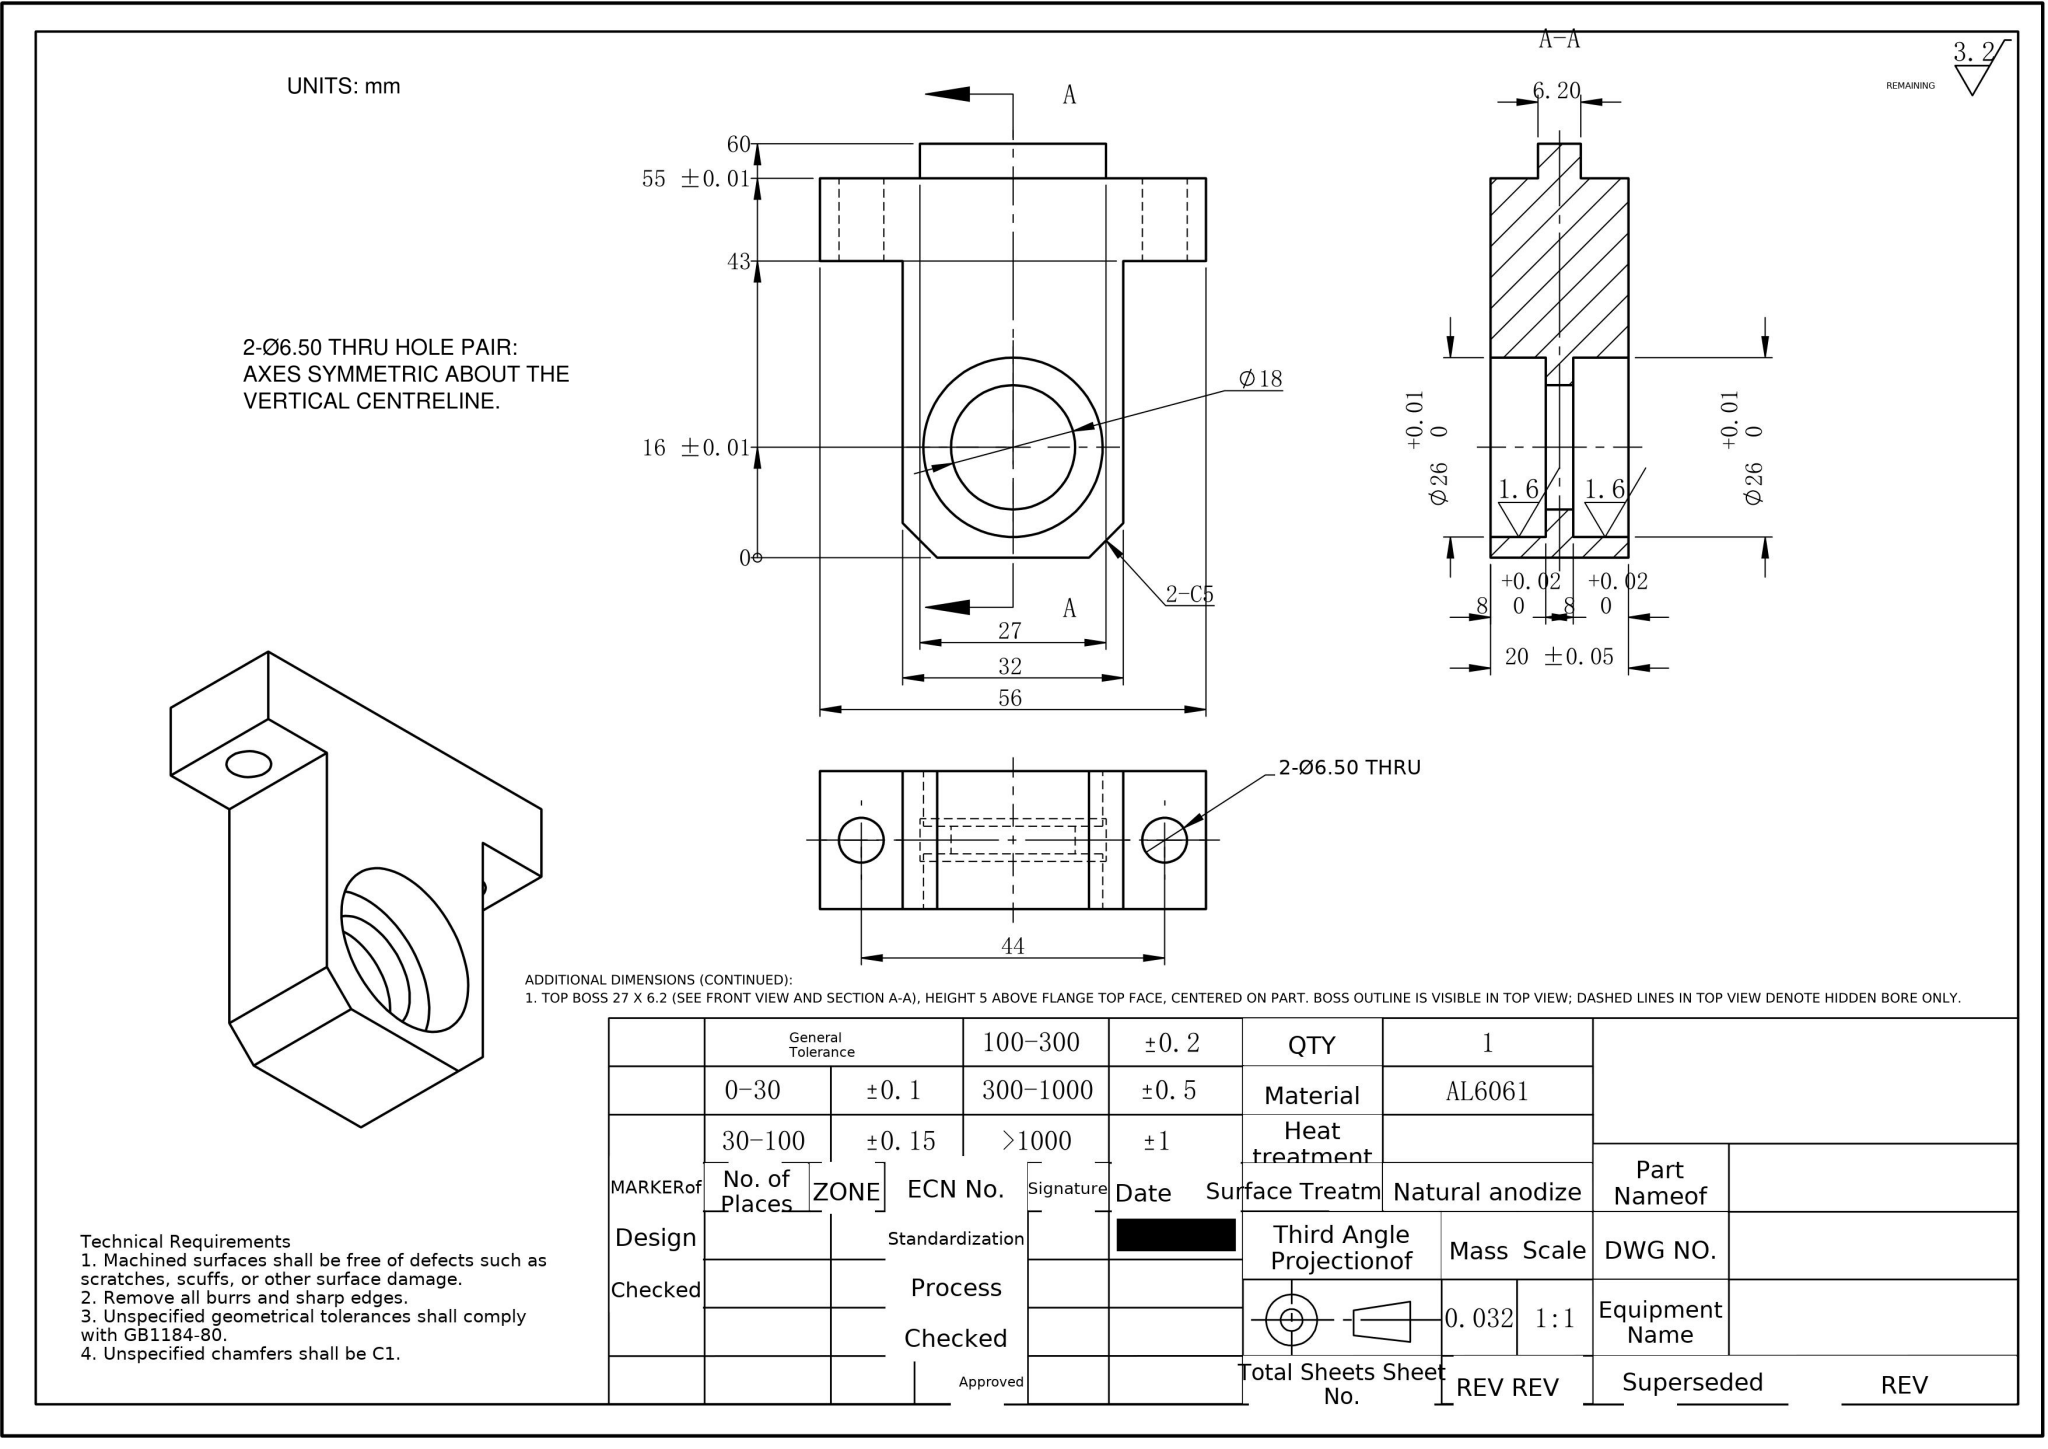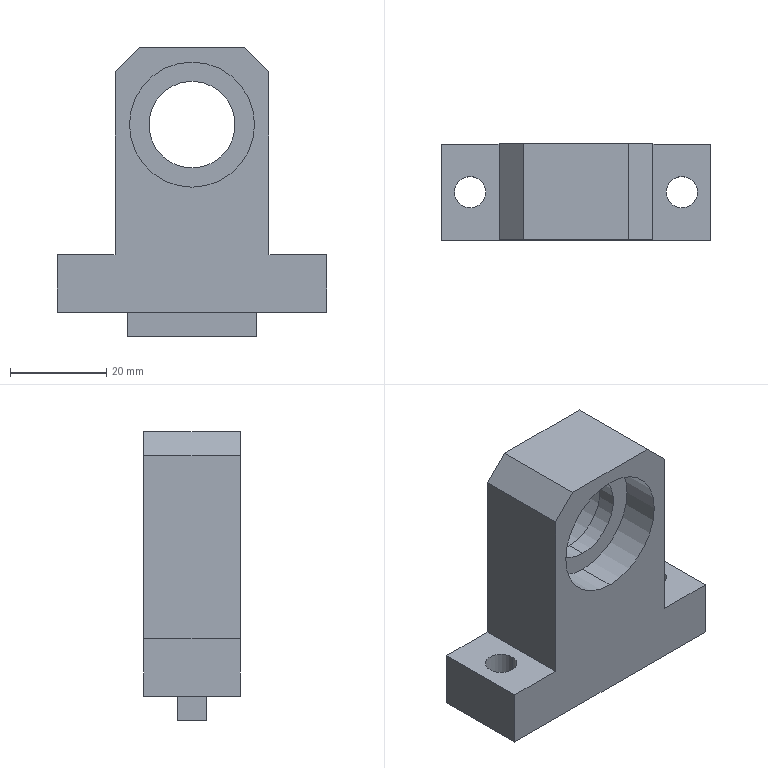Part | NX | mm | 1 solid | 29 faces | box 56 x 20 x 60 mm | volume 30988 mm3 | plane 19 | cylinder 10 | commonest cylinder face diameters 26 x4 6.5 x4 18 x2
STEP:
#1=CARTESIAN_POINT('',(0.,2.,-28.75));
#2=VERTEX_POINT('',#1);
#3=CARTESIAN_POINT('',(0.,2.,-54.75));
#4=VERTEX_POINT('',#3);
#5=CARTESIAN_POINT('',(0.,2.,-41.75));
#6=DIRECTION('',(0.,-1.,0.));
#7=DIRECTION('',(0.,0.,-1.));
#8=AXIS2_PLACEMENT_3D('',#5,#6,#7);
#9=CIRCLE('',#8,13.);
#10=EDGE_CURVE('',#2,#4,#9,.T.);
#11=ORIENTED_EDGE('',*,*,#10,.T.);
#12=CARTESIAN_POINT('',(0.,10.,-54.75));
#13=VERTEX_POINT('',#12);
#14=CARTESIAN_POINT('',(0.,2.,-54.75));
#15=DIRECTION('',(0.,1.,0.));
#16=VECTOR('',#15,1000.);
#17=LINE('',#14,#16);
#18=EDGE_CURVE('',#4,#13,#17,.T.);
#19=ORIENTED_EDGE('',*,*,#18,.T.);
#20=CARTESIAN_POINT('',(0.,10.,-28.75));
#21=VERTEX_POINT('',#20);
#22=CARTESIAN_POINT('',(0.,10.,-41.75));
#23=DIRECTION('',(0.,-1.,0.));
#24=DIRECTION('',(0.,0.,-1.));
#25=AXIS2_PLACEMENT_3D('',#22,#23,#24);
#26=CIRCLE('',#25,13.);
#27=EDGE_CURVE('',#21,#13,#26,.T.);
#28=ORIENTED_EDGE('',*,*,#27,.F.);
#29=CARTESIAN_POINT('',(0.,2.,-28.75));
#30=DIRECTION('',(0.,1.,0.));
#31=VECTOR('',#30,1000.);
#32=LINE('',#29,#31);
#33=EDGE_CURVE('',#2,#21,#32,.T.);
#34=ORIENTED_EDGE('',*,*,#33,.F.);
#35=EDGE_LOOP('',(#11,#19,#28,#34));
#36=FACE_OUTER_BOUND('',#35,.T.);
#37=CARTESIAN_POINT('',(0.,2.,-41.75));
#38=DIRECTION('',(0.,1.,0.));
#39=DIRECTION('',(0.,0.,1.));
#40=AXIS2_PLACEMENT_3D('',#37,#38,#39);
#41=CYLINDRICAL_SURFACE('',#40,13.);
#42=ADVANCED_FACE('',(#36),#41,.F.);
#43=CARTESIAN_POINT('',(0.,-2.,-28.75));
#44=VERTEX_POINT('',#43);
#45=CARTESIAN_POINT('',(0.,-2.,-54.75));
#46=VERTEX_POINT('',#45);
#47=CARTESIAN_POINT('',(0.,-2.,-41.75));
#48=DIRECTION('',(0.,-1.,0.));
#49=DIRECTION('',(0.,0.,-1.));
#50=AXIS2_PLACEMENT_3D('',#47,#48,#49);
#51=CIRCLE('',#50,13.);
#52=EDGE_CURVE('',#44,#46,#51,.T.);
#53=ORIENTED_EDGE('',*,*,#52,.F.);
#54=CARTESIAN_POINT('',(0.,-10.,-28.75));
#55=VERTEX_POINT('',#54);
#56=CARTESIAN_POINT('',(0.,-2.,-28.75));
#57=DIRECTION('',(0.,-1.,0.));
#58=VECTOR('',#57,1000.);
#59=LINE('',#56,#58);
#60=EDGE_CURVE('',#44,#55,#59,.T.);
#61=ORIENTED_EDGE('',*,*,#60,.T.);
#62=CARTESIAN_POINT('',(0.,-10.,-54.75));
#63=VERTEX_POINT('',#62);
#64=CARTESIAN_POINT('',(0.,-10.,-41.75));
#65=DIRECTION('',(0.,-1.,0.));
#66=DIRECTION('',(0.,0.,-1.));
#67=AXIS2_PLACEMENT_3D('',#64,#65,#66);
#68=CIRCLE('',#67,13.);
#69=EDGE_CURVE('',#55,#63,#68,.T.);
#70=ORIENTED_EDGE('',*,*,#69,.T.);
#71=CARTESIAN_POINT('',(0.,-2.,-54.75));
#72=DIRECTION('',(0.,-1.,0.));
#73=VECTOR('',#72,1000.);
#74=LINE('',#71,#73);
#75=EDGE_CURVE('',#46,#63,#74,.T.);
#76=ORIENTED_EDGE('',*,*,#75,.F.);
#77=EDGE_LOOP('',(#53,#61,#70,#76));
#78=FACE_OUTER_BOUND('',#77,.T.);
#79=CARTESIAN_POINT('',(0.,-2.,-41.75));
#80=DIRECTION('',(0.,-1.,0.));
#81=DIRECTION('',(0.,0.,-1.));
#82=AXIS2_PLACEMENT_3D('',#79,#80,#81);
#83=CYLINDRICAL_SURFACE('',#82,13.);
#84=ADVANCED_FACE('',(#78),#83,.F.);
#85=CARTESIAN_POINT('',(25.25,-0.,-68.75));
#86=VERTEX_POINT('',#85);
#87=CARTESIAN_POINT('',(18.75,-0.,-68.75));
#88=VERTEX_POINT('',#87);
#89=CARTESIAN_POINT('',(22.,-0.,-68.75));
#90=DIRECTION('',(0.,0.,-1.));
#91=DIRECTION('',(-1.,0.,0.));
#92=AXIS2_PLACEMENT_3D('',#89,#90,#91);
#93=CIRCLE('',#92,3.25);
#94=EDGE_CURVE('',#86,#88,#93,.T.);
#95=ORIENTED_EDGE('',*,*,#94,.F.);
#96=CARTESIAN_POINT('',(25.25,-0.,-80.75));
#97=VERTEX_POINT('',#96);
#98=CARTESIAN_POINT('',(25.25,-0.,89.942));
#99=DIRECTION('',(0.,0.,-1.));
#100=VECTOR('',#99,1000.);
#101=LINE('',#98,#100);
#102=EDGE_CURVE('',#86,#97,#101,.T.);
#103=ORIENTED_EDGE('',*,*,#102,.T.);
#104=CARTESIAN_POINT('',(18.75,-0.,-80.75));
#105=VERTEX_POINT('',#104);
#106=CARTESIAN_POINT('',(22.,-0.,-80.75));
#107=DIRECTION('',(0.,0.,-1.));
#108=DIRECTION('',(1.,0.,0.));
#109=AXIS2_PLACEMENT_3D('',#106,#107,#108);
#110=CIRCLE('',#109,3.25);
#111=EDGE_CURVE('',#97,#105,#110,.T.);
#112=ORIENTED_EDGE('',*,*,#111,.T.);
#113=CARTESIAN_POINT('',(18.75,-0.,89.942));
#114=DIRECTION('',(0.,0.,-1.));
#115=VECTOR('',#114,1000.);
#116=LINE('',#113,#115);
#117=EDGE_CURVE('',#88,#105,#116,.T.);
#118=ORIENTED_EDGE('',*,*,#117,.F.);
#119=EDGE_LOOP('',(#95,#103,#112,#118));
#120=FACE_OUTER_BOUND('',#119,.T.);
#121=CARTESIAN_POINT('',(22.,-0.,89.942));
#122=DIRECTION('',(0.,0.,-1.));
#123=DIRECTION('',(-1.,0.,0.));
#124=AXIS2_PLACEMENT_3D('',#121,#122,#123);
#125=CYLINDRICAL_SURFACE('',#124,3.25);
#126=ADVANCED_FACE('',(#120),#125,.F.);
#127=CARTESIAN_POINT('',(-18.75,0.,-68.75));
#128=VERTEX_POINT('',#127);
#129=CARTESIAN_POINT('',(-25.25,0.,-68.75));
#130=VERTEX_POINT('',#129);
#131=CARTESIAN_POINT('',(-22.,0.,-68.75));
#132=DIRECTION('',(0.,0.,-1.));
#133=DIRECTION('',(-1.,0.,0.));
#134=AXIS2_PLACEMENT_3D('',#131,#132,#133);
#135=CIRCLE('',#134,3.25);
#136=EDGE_CURVE('',#128,#130,#135,.T.);
#137=ORIENTED_EDGE('',*,*,#136,.F.);
#138=CARTESIAN_POINT('',(-18.75,0.,-80.75));
#139=VERTEX_POINT('',#138);
#140=CARTESIAN_POINT('',(-18.75,0.,89.942));
#141=DIRECTION('',(0.,0.,-1.));
#142=VECTOR('',#141,1000.);
#143=LINE('',#140,#142);
#144=EDGE_CURVE('',#128,#139,#143,.T.);
#145=ORIENTED_EDGE('',*,*,#144,.T.);
#146=CARTESIAN_POINT('',(-25.25,0.,-80.75));
#147=VERTEX_POINT('',#146);
#148=CARTESIAN_POINT('',(-22.,0.,-80.75));
#149=DIRECTION('',(0.,0.,-1.));
#150=DIRECTION('',(-1.,0.,0.));
#151=AXIS2_PLACEMENT_3D('',#148,#149,#150);
#152=CIRCLE('',#151,3.25);
#153=EDGE_CURVE('',#139,#147,#152,.T.);
#154=ORIENTED_EDGE('',*,*,#153,.T.);
#155=CARTESIAN_POINT('',(-25.25,0.,89.942));
#156=DIRECTION('',(0.,0.,-1.));
#157=VECTOR('',#156,1000.);
#158=LINE('',#155,#157);
#159=EDGE_CURVE('',#130,#147,#158,.T.);
#160=ORIENTED_EDGE('',*,*,#159,.F.);
#161=EDGE_LOOP('',(#137,#145,#154,#160));
#162=FACE_OUTER_BOUND('',#161,.T.);
#163=CARTESIAN_POINT('',(-22.,0.,89.942));
#164=DIRECTION('',(0.,0.,-1.));
#165=DIRECTION('',(-1.,0.,0.));
#166=AXIS2_PLACEMENT_3D('',#163,#164,#165);
#167=CYLINDRICAL_SURFACE('',#166,3.25);
#168=ADVANCED_FACE('',(#162),#167,.F.);
#169=CARTESIAN_POINT('',(0.,2.,-32.75));
#170=VERTEX_POINT('',#169);
#171=CARTESIAN_POINT('',(0.,2.,-50.75));
#172=VERTEX_POINT('',#171);
#173=CARTESIAN_POINT('',(0.,2.,-41.75));
#174=DIRECTION('',(0.,-1.,0.));
#175=DIRECTION('',(0.,0.,1.));
#176=AXIS2_PLACEMENT_3D('',#173,#174,#175);
#177=CIRCLE('',#176,9.);
#178=EDGE_CURVE('',#170,#172,#177,.T.);
#179=ORIENTED_EDGE('',*,*,#178,.F.);
#180=CARTESIAN_POINT('',(0.,-2.,-32.75));
#181=VERTEX_POINT('',#180);
#182=CARTESIAN_POINT('',(0.,11.,-32.75));
#183=DIRECTION('',(0.,-1.,0.));
#184=VECTOR('',#183,1000.);
#185=LINE('',#182,#184);
#186=EDGE_CURVE('',#170,#181,#185,.T.);
#187=ORIENTED_EDGE('',*,*,#186,.T.);
#188=CARTESIAN_POINT('',(0.,-2.,-50.75));
#189=VERTEX_POINT('',#188);
#190=CARTESIAN_POINT('',(0.,-2.,-41.75));
#191=DIRECTION('',(0.,1.,0.));
#192=DIRECTION('',(0.,0.,-1.));
#193=AXIS2_PLACEMENT_3D('',#190,#191,#192);
#194=CIRCLE('',#193,9.);
#195=EDGE_CURVE('',#189,#181,#194,.T.);
#196=ORIENTED_EDGE('',*,*,#195,.F.);
#197=CARTESIAN_POINT('',(0.,11.,-50.75));
#198=DIRECTION('',(0.,-1.,0.));
#199=VECTOR('',#198,1000.);
#200=LINE('',#197,#199);
#201=EDGE_CURVE('',#172,#189,#200,.T.);
#202=ORIENTED_EDGE('',*,*,#201,.F.);
#203=EDGE_LOOP('',(#179,#187,#196,#202));
#204=FACE_OUTER_BOUND('',#203,.T.);
#205=CARTESIAN_POINT('',(0.,11.,-41.75));
#206=DIRECTION('',(0.,-1.,0.));
#207=DIRECTION('',(0.,0.,-1.));
#208=AXIS2_PLACEMENT_3D('',#205,#206,#207);
#209=CYLINDRICAL_SURFACE('',#208,9.);
#210=ADVANCED_FACE('',(#204),#209,.F.);
#211=ORIENTED_EDGE('',*,*,#186,.F.);
#212=CARTESIAN_POINT('',(0.,2.,-41.75));
#213=DIRECTION('',(0.,-1.,0.));
#214=DIRECTION('',(0.,0.,1.));
#215=AXIS2_PLACEMENT_3D('',#212,#213,#214);
#216=CIRCLE('',#215,9.);
#217=EDGE_CURVE('',#172,#170,#216,.T.);
#218=ORIENTED_EDGE('',*,*,#217,.F.);
#219=ORIENTED_EDGE('',*,*,#201,.T.);
#220=CARTESIAN_POINT('',(0.,-2.,-41.75));
#221=DIRECTION('',(0.,1.,0.));
#222=DIRECTION('',(0.,0.,-1.));
#223=AXIS2_PLACEMENT_3D('',#220,#221,#222);
#224=CIRCLE('',#223,9.);
#225=EDGE_CURVE('',#181,#189,#224,.T.);
#226=ORIENTED_EDGE('',*,*,#225,.F.);
#227=EDGE_LOOP('',(#211,#218,#219,#226));
#228=FACE_OUTER_BOUND('',#227,.T.);
#229=CARTESIAN_POINT('',(0.,11.,-41.75));
#230=DIRECTION('',(0.,-1.,0.));
#231=DIRECTION('',(0.,0.,-1.));
#232=AXIS2_PLACEMENT_3D('',#229,#230,#231);
#233=CYLINDRICAL_SURFACE('',#232,9.);
#234=ADVANCED_FACE('',(#228),#233,.F.);
#235=CARTESIAN_POINT('',(-16.,10.,-68.75));
#236=VERTEX_POINT('',#235);
#237=CARTESIAN_POINT('',(-16.,10.,-30.75));
#238=VERTEX_POINT('',#237);
#239=CARTESIAN_POINT('',(-16.,10.,-68.75));
#240=DIRECTION('',(0.,0.,1.));
#241=VECTOR('',#240,1000.);
#242=LINE('',#239,#241);
#243=EDGE_CURVE('',#236,#238,#242,.T.);
#244=ORIENTED_EDGE('',*,*,#243,.T.);
#245=CARTESIAN_POINT('',(-11.,10.,-25.75));
#246=VERTEX_POINT('',#245);
#247=CARTESIAN_POINT('',(-16.,10.,-30.75));
#248=DIRECTION('',(0.7071,0.,0.7071));
#249=VECTOR('',#248,1000.);
#250=LINE('',#247,#249);
#251=EDGE_CURVE('',#238,#246,#250,.T.);
#252=ORIENTED_EDGE('',*,*,#251,.T.);
#253=CARTESIAN_POINT('',(11.,10.,-25.75));
#254=VERTEX_POINT('',#253);
#255=CARTESIAN_POINT('',(0.,10.,-25.75));
#256=DIRECTION('',(1.,0.,0.));
#257=VECTOR('',#256,1000.);
#258=LINE('',#255,#257);
#259=EDGE_CURVE('',#246,#254,#258,.T.);
#260=ORIENTED_EDGE('',*,*,#259,.T.);
#261=CARTESIAN_POINT('',(16.,10.,-30.75));
#262=VERTEX_POINT('',#261);
#263=CARTESIAN_POINT('',(16.,10.,-30.75));
#264=DIRECTION('',(0.7071,0.,-0.7071));
#265=VECTOR('',#264,1000.);
#266=LINE('',#263,#265);
#267=EDGE_CURVE('',#254,#262,#266,.T.);
#268=ORIENTED_EDGE('',*,*,#267,.T.);
#269=CARTESIAN_POINT('',(16.,10.,-68.75));
#270=VERTEX_POINT('',#269);
#271=CARTESIAN_POINT('',(16.,10.,-68.75));
#272=DIRECTION('',(0.,0.,-1.));
#273=VECTOR('',#272,1000.);
#274=LINE('',#271,#273);
#275=EDGE_CURVE('',#262,#270,#274,.T.);
#276=ORIENTED_EDGE('',*,*,#275,.T.);
#277=CARTESIAN_POINT('',(28.,10.,-68.75));
#278=VERTEX_POINT('',#277);
#279=CARTESIAN_POINT('',(28.,10.,-68.75));
#280=DIRECTION('',(1.,0.,0.));
#281=VECTOR('',#280,1000.);
#282=LINE('',#279,#281);
#283=EDGE_CURVE('',#270,#278,#282,.T.);
#284=ORIENTED_EDGE('',*,*,#283,.T.);
#285=CARTESIAN_POINT('',(28.,10.,-80.75));
#286=VERTEX_POINT('',#285);
#287=CARTESIAN_POINT('',(28.,10.,80.75));
#288=DIRECTION('',(0.,0.,-1.));
#289=VECTOR('',#288,1000.);
#290=LINE('',#287,#289);
#291=EDGE_CURVE('',#278,#286,#290,.T.);
#292=ORIENTED_EDGE('',*,*,#291,.T.);
#293=CARTESIAN_POINT('',(-28.,10.,-80.75));
#294=VERTEX_POINT('',#293);
#295=CARTESIAN_POINT('',(-28.,10.,-80.75));
#296=DIRECTION('',(-1.,0.,0.));
#297=VECTOR('',#296,1000.);
#298=LINE('',#295,#297);
#299=EDGE_CURVE('',#286,#294,#298,.T.);
#300=ORIENTED_EDGE('',*,*,#299,.T.);
#301=CARTESIAN_POINT('',(-28.,10.,-68.75));
#302=VERTEX_POINT('',#301);
#303=CARTESIAN_POINT('',(-28.,10.,80.75));
#304=DIRECTION('',(0.,0.,1.));
#305=VECTOR('',#304,1000.);
#306=LINE('',#303,#305);
#307=EDGE_CURVE('',#294,#302,#306,.T.);
#308=ORIENTED_EDGE('',*,*,#307,.T.);
#309=CARTESIAN_POINT('',(-28.,10.,-68.75));
#310=DIRECTION('',(1.,0.,0.));
#311=VECTOR('',#310,1000.);
#312=LINE('',#309,#311);
#313=EDGE_CURVE('',#302,#236,#312,.T.);
#314=ORIENTED_EDGE('',*,*,#313,.T.);
#315=EDGE_LOOP('',(#244,#252,#260,#268,#276,#284,#292,#300,#308,#314));
#316=FACE_OUTER_BOUND('',#315,.T.);
#317=ORIENTED_EDGE('',*,*,#27,.T.);
#318=CARTESIAN_POINT('',(0.,10.,-41.75));
#319=DIRECTION('',(0.,-1.,0.));
#320=DIRECTION('',(0.,0.,-1.));
#321=AXIS2_PLACEMENT_3D('',#318,#319,#320);
#322=CIRCLE('',#321,13.);
#323=EDGE_CURVE('',#13,#21,#322,.T.);
#324=ORIENTED_EDGE('',*,*,#323,.T.);
#325=EDGE_LOOP('',(#317,#324));
#326=FACE_BOUND('',#325,.T.);
#327=CARTESIAN_POINT('',(0.,10.,0.));
#328=DIRECTION('',(0.,-1.,0.));
#329=DIRECTION('',(0.,0.,-1.));
#330=AXIS2_PLACEMENT_3D('',#327,#328,#329);
#331=PLANE('',#330);
#332=ADVANCED_FACE('',(#316,#326),#331,.F.);
#333=CARTESIAN_POINT('',(22.,-0.,-80.75));
#334=DIRECTION('',(0.,0.,-1.));
#335=DIRECTION('',(1.,0.,0.));
#336=AXIS2_PLACEMENT_3D('',#333,#334,#335);
#337=CIRCLE('',#336,3.25);
#338=EDGE_CURVE('',#105,#97,#337,.T.);
#339=ORIENTED_EDGE('',*,*,#338,.F.);
#340=ORIENTED_EDGE('',*,*,#111,.F.);
#341=EDGE_LOOP('',(#339,#340));
#342=FACE_BOUND('',#341,.T.);
#343=CARTESIAN_POINT('',(-22.,0.,-80.75));
#344=DIRECTION('',(0.,0.,-1.));
#345=DIRECTION('',(-1.,0.,0.));
#346=AXIS2_PLACEMENT_3D('',#343,#344,#345);
#347=CIRCLE('',#346,3.25);
#348=EDGE_CURVE('',#147,#139,#347,.T.);
#349=ORIENTED_EDGE('',*,*,#348,.F.);
#350=ORIENTED_EDGE('',*,*,#153,.F.);
#351=EDGE_LOOP('',(#349,#350));
#352=FACE_BOUND('',#351,.T.);
#353=CARTESIAN_POINT('',(28.,-10.,-80.75));
#354=VERTEX_POINT('',#353);
#355=CARTESIAN_POINT('',(-28.,-10.,-80.75));
#356=VERTEX_POINT('',#355);
#357=CARTESIAN_POINT('',(-28.,-10.,-80.75));
#358=DIRECTION('',(-1.,0.,0.));
#359=VECTOR('',#358,1000.);
#360=LINE('',#357,#359);
#361=EDGE_CURVE('',#354,#356,#360,.T.);
#362=ORIENTED_EDGE('',*,*,#361,.T.);
#363=CARTESIAN_POINT('',(-28.,10.,-80.75));
#364=DIRECTION('',(0.,-1.,0.));
#365=VECTOR('',#364,1000.);
#366=LINE('',#363,#365);
#367=EDGE_CURVE('',#294,#356,#366,.T.);
#368=ORIENTED_EDGE('',*,*,#367,.F.);
#369=ORIENTED_EDGE('',*,*,#299,.F.);
#370=CARTESIAN_POINT('',(28.,10.,-80.75));
#371=DIRECTION('',(0.,-1.,0.));
#372=VECTOR('',#371,1000.);
#373=LINE('',#370,#372);
#374=EDGE_CURVE('',#286,#354,#373,.T.);
#375=ORIENTED_EDGE('',*,*,#374,.T.);
#376=EDGE_LOOP('',(#362,#368,#369,#375));
#377=FACE_OUTER_BOUND('',#376,.T.);
#378=CARTESIAN_POINT('',(-13.5,-3.1,-80.75));
#379=VERTEX_POINT('',#378);
#380=CARTESIAN_POINT('',(-13.5,3.1,-80.75));
#381=VERTEX_POINT('',#380);
#382=CARTESIAN_POINT('',(-13.5,-3.1,-80.75));
#383=DIRECTION('',(0.,1.,0.));
#384=VECTOR('',#383,1000.);
#385=LINE('',#382,#384);
#386=EDGE_CURVE('',#379,#381,#385,.T.);
#387=ORIENTED_EDGE('',*,*,#386,.F.);
#388=CARTESIAN_POINT('',(13.5,-3.1,-80.75));
#389=VERTEX_POINT('',#388);
#390=CARTESIAN_POINT('',(13.5,-3.1,-80.75));
#391=DIRECTION('',(-1.,0.,0.));
#392=VECTOR('',#391,1000.);
#393=LINE('',#390,#392);
#394=EDGE_CURVE('',#389,#379,#393,.T.);
#395=ORIENTED_EDGE('',*,*,#394,.F.);
#396=CARTESIAN_POINT('',(13.5,3.1,-80.75));
#397=VERTEX_POINT('',#396);
#398=CARTESIAN_POINT('',(13.5,-3.1,-80.75));
#399=DIRECTION('',(0.,-1.,0.));
#400=VECTOR('',#399,1000.);
#401=LINE('',#398,#400);
#402=EDGE_CURVE('',#397,#389,#401,.T.);
#403=ORIENTED_EDGE('',*,*,#402,.F.);
#404=CARTESIAN_POINT('',(13.5,3.1,-80.75));
#405=DIRECTION('',(1.,0.,0.));
#406=VECTOR('',#405,1000.);
#407=LINE('',#404,#406);
#408=EDGE_CURVE('',#381,#397,#407,.T.);
#409=ORIENTED_EDGE('',*,*,#408,.F.);
#410=EDGE_LOOP('',(#387,#395,#403,#409));
#411=FACE_BOUND('',#410,.T.);
#412=CARTESIAN_POINT('',(-28.,10.,-80.75));
#413=DIRECTION('',(0.,0.,1.));
#414=DIRECTION('',(1.,0.,0.));
#415=AXIS2_PLACEMENT_3D('',#412,#413,#414);
#416=PLANE('',#415);
#417=ADVANCED_FACE('',(#342,#352,#377,#411),#416,.F.);
#418=ORIENTED_EDGE('',*,*,#291,.F.);
#419=CARTESIAN_POINT('',(28.,-10.,-68.75));
#420=VERTEX_POINT('',#419);
#421=CARTESIAN_POINT('',(28.,10.,-68.75));
#422=DIRECTION('',(0.,-1.,0.));
#423=VECTOR('',#422,1000.);
#424=LINE('',#421,#423);
#425=EDGE_CURVE('',#278,#420,#424,.T.);
#426=ORIENTED_EDGE('',*,*,#425,.T.);
#427=CARTESIAN_POINT('',(28.,-10.,80.75));
#428=DIRECTION('',(0.,0.,-1.));
#429=VECTOR('',#428,1000.);
#430=LINE('',#427,#429);
#431=EDGE_CURVE('',#420,#354,#430,.T.);
#432=ORIENTED_EDGE('',*,*,#431,.T.);
#433=ORIENTED_EDGE('',*,*,#374,.F.);
#434=EDGE_LOOP('',(#418,#426,#432,#433));
#435=FACE_OUTER_BOUND('',#434,.T.);
#436=CARTESIAN_POINT('',(28.,10.,80.75));
#437=DIRECTION('',(-1.,0.,0.));
#438=DIRECTION('',(0.,0.,1.));
#439=AXIS2_PLACEMENT_3D('',#436,#437,#438);
#440=PLANE('',#439);
#441=ADVANCED_FACE('',(#435),#440,.F.);
#442=CARTESIAN_POINT('',(-28.,-10.,-68.75));
#443=VERTEX_POINT('',#442);
#444=CARTESIAN_POINT('',(-28.,-10.,80.75));
#445=DIRECTION('',(0.,0.,1.));
#446=VECTOR('',#445,1000.);
#447=LINE('',#444,#446);
#448=EDGE_CURVE('',#356,#443,#447,.T.);
#449=ORIENTED_EDGE('',*,*,#448,.T.);
#450=CARTESIAN_POINT('',(-28.,10.,-68.75));
#451=DIRECTION('',(0.,-1.,0.));
#452=VECTOR('',#451,1000.);
#453=LINE('',#450,#452);
#454=EDGE_CURVE('',#302,#443,#453,.T.);
#455=ORIENTED_EDGE('',*,*,#454,.F.);
#456=ORIENTED_EDGE('',*,*,#307,.F.);
#457=ORIENTED_EDGE('',*,*,#367,.T.);
#458=EDGE_LOOP('',(#449,#455,#456,#457));
#459=FACE_OUTER_BOUND('',#458,.T.);
#460=CARTESIAN_POINT('',(-28.,10.,80.75));
#461=DIRECTION('',(1.,0.,0.));
#462=DIRECTION('',(0.,0.,-1.));
#463=AXIS2_PLACEMENT_3D('',#460,#461,#462);
#464=PLANE('',#463);
#465=ADVANCED_FACE('',(#459),#464,.F.);
#466=CARTESIAN_POINT('',(0.,-10.,-41.75));
#467=DIRECTION('',(0.,-1.,0.));
#468=DIRECTION('',(0.,0.,-1.));
#469=AXIS2_PLACEMENT_3D('',#466,#467,#468);
#470=CIRCLE('',#469,13.);
#471=EDGE_CURVE('',#63,#55,#470,.T.);
#472=ORIENTED_EDGE('',*,*,#471,.F.);
#473=ORIENTED_EDGE('',*,*,#69,.F.);
#474=EDGE_LOOP('',(#472,#473));
#475=FACE_BOUND('',#474,.T.);
#476=CARTESIAN_POINT('',(-11.,-10.,-25.75));
#477=VERTEX_POINT('',#476);
#478=CARTESIAN_POINT('',(11.,-10.,-25.75));
#479=VERTEX_POINT('',#478);
#480=CARTESIAN_POINT('',(-28.,-10.,-25.75));
#481=DIRECTION('',(1.,0.,0.));
#482=VECTOR('',#481,1000.);
#483=LINE('',#480,#482);
#484=EDGE_CURVE('',#477,#479,#483,.T.);
#485=ORIENTED_EDGE('',*,*,#484,.F.);
#486=CARTESIAN_POINT('',(-16.,-10.,-30.75));
#487=VERTEX_POINT('',#486);
#488=CARTESIAN_POINT('',(7.375,-10.,-7.375));
#489=DIRECTION('',(-0.7071,0.,-0.7071));
#490=VECTOR('',#489,1000.);
#491=LINE('',#488,#490);
#492=EDGE_CURVE('',#477,#487,#491,.T.);
#493=ORIENTED_EDGE('',*,*,#492,.T.);
#494=CARTESIAN_POINT('',(-16.,-10.,-68.75));
#495=VERTEX_POINT('',#494);
#496=CARTESIAN_POINT('',(-16.,-10.,-68.75));
#497=DIRECTION('',(0.,0.,1.));
#498=VECTOR('',#497,1000.);
#499=LINE('',#496,#498);
#500=EDGE_CURVE('',#495,#487,#499,.T.);
#501=ORIENTED_EDGE('',*,*,#500,.F.);
#502=CARTESIAN_POINT('',(-28.,-10.,-68.75));
#503=DIRECTION('',(1.,0.,0.));
#504=VECTOR('',#503,1000.);
#505=LINE('',#502,#504);
#506=EDGE_CURVE('',#443,#495,#505,.T.);
#507=ORIENTED_EDGE('',*,*,#506,.F.);
#508=ORIENTED_EDGE('',*,*,#448,.F.);
#509=ORIENTED_EDGE('',*,*,#361,.F.);
#510=ORIENTED_EDGE('',*,*,#431,.F.);
#511=CARTESIAN_POINT('',(16.,-10.,-68.75));
#512=VERTEX_POINT('',#511);
#513=CARTESIAN_POINT('',(28.,-10.,-68.75));
#514=DIRECTION('',(1.,0.,0.));
#515=VECTOR('',#514,1000.);
#516=LINE('',#513,#515);
#517=EDGE_CURVE('',#512,#420,#516,.T.);
#518=ORIENTED_EDGE('',*,*,#517,.F.);
#519=CARTESIAN_POINT('',(16.,-10.,-30.75));
#520=VERTEX_POINT('',#519);
#521=CARTESIAN_POINT('',(16.,-10.,-68.75));
#522=DIRECTION('',(0.,0.,-1.));
#523=VECTOR('',#522,1000.);
#524=LINE('',#521,#523);
#525=EDGE_CURVE('',#520,#512,#524,.T.);
#526=ORIENTED_EDGE('',*,*,#525,.F.);
#527=CARTESIAN_POINT('',(-7.375,-10.,-7.375));
#528=DIRECTION('',(-0.7071,0.,0.7071));
#529=VECTOR('',#528,1000.);
#530=LINE('',#527,#529);
#531=EDGE_CURVE('',#520,#479,#530,.T.);
#532=ORIENTED_EDGE('',*,*,#531,.T.);
#533=EDGE_LOOP('',(#485,#493,#501,#507,#508,#509,#510,#518,#526,#532));
#534=FACE_OUTER_BOUND('',#533,.T.);
#535=CARTESIAN_POINT('',(0.,-10.,0.));
#536=DIRECTION('',(0.,-1.,0.));
#537=DIRECTION('',(0.,0.,-1.));
#538=AXIS2_PLACEMENT_3D('',#535,#536,#537);
#539=PLANE('',#538);
#540=ADVANCED_FACE('',(#475,#534),#539,.T.);
#541=ORIENTED_EDGE('',*,*,#500,.T.);
#542=CARTESIAN_POINT('',(-16.,10.,-30.75));
#543=DIRECTION('',(0.,1.,0.));
#544=VECTOR('',#543,1000.);
#545=LINE('',#542,#544);
#546=EDGE_CURVE('',#487,#238,#545,.T.);
#547=ORIENTED_EDGE('',*,*,#546,.T.);
#548=ORIENTED_EDGE('',*,*,#243,.F.);
#549=CARTESIAN_POINT('',(-16.,10.,-68.75));
#550=DIRECTION('',(0.,-1.,0.));
#551=VECTOR('',#550,1000.);
#552=LINE('',#549,#551);
#553=EDGE_CURVE('',#236,#495,#552,.T.);
#554=ORIENTED_EDGE('',*,*,#553,.T.);
#555=EDGE_LOOP('',(#541,#547,#548,#554));
#556=FACE_OUTER_BOUND('',#555,.T.);
#557=CARTESIAN_POINT('',(-16.,10.,-68.75));
#558=DIRECTION('',(1.,0.,0.));
#559=DIRECTION('',(0.,0.,-1.));
#560=AXIS2_PLACEMENT_3D('',#557,#558,#559);
#561=PLANE('',#560);
#562=ADVANCED_FACE('',(#556),#561,.F.);
#563=CARTESIAN_POINT('',(-22.,0.,-68.75));
#564=DIRECTION('',(0.,0.,-1.));
#565=DIRECTION('',(-1.,0.,0.));
#566=AXIS2_PLACEMENT_3D('',#563,#564,#565);
#567=CIRCLE('',#566,3.25);
#568=EDGE_CURVE('',#130,#128,#567,.T.);
#569=ORIENTED_EDGE('',*,*,#568,.T.);
#570=ORIENTED_EDGE('',*,*,#136,.T.);
#571=EDGE_LOOP('',(#569,#570));
#572=FACE_BOUND('',#571,.T.);
#573=ORIENTED_EDGE('',*,*,#506,.T.);
#574=ORIENTED_EDGE('',*,*,#553,.F.);
#575=ORIENTED_EDGE('',*,*,#313,.F.);
#576=ORIENTED_EDGE('',*,*,#454,.T.);
#577=EDGE_LOOP('',(#573,#574,#575,#576));
#578=FACE_OUTER_BOUND('',#577,.T.);
#579=CARTESIAN_POINT('',(-28.,10.,-68.75));
#580=DIRECTION('',(0.,0.,-1.));
#581=DIRECTION('',(-1.,0.,0.));
#582=AXIS2_PLACEMENT_3D('',#579,#580,#581);
#583=PLANE('',#582);
#584=ADVANCED_FACE('',(#572,#578),#583,.F.);
#585=CARTESIAN_POINT('',(22.,-0.,-68.75));
#586=DIRECTION('',(0.,0.,-1.));
#587=DIRECTION('',(-1.,0.,0.));
#588=AXIS2_PLACEMENT_3D('',#585,#586,#587);
#589=CIRCLE('',#588,3.25);
#590=EDGE_CURVE('',#88,#86,#589,.T.);
#591=ORIENTED_EDGE('',*,*,#590,.T.);
#592=ORIENTED_EDGE('',*,*,#94,.T.);
#593=EDGE_LOOP('',(#591,#592));
#594=FACE_BOUND('',#593,.T.);
#595=ORIENTED_EDGE('',*,*,#517,.T.);
#596=ORIENTED_EDGE('',*,*,#425,.F.);
#597=ORIENTED_EDGE('',*,*,#283,.F.);
#598=CARTESIAN_POINT('',(16.,10.,-68.75));
#599=DIRECTION('',(0.,-1.,0.));
#600=VECTOR('',#599,1000.);
#601=LINE('',#598,#600);
#602=EDGE_CURVE('',#270,#512,#601,.T.);
#603=ORIENTED_EDGE('',*,*,#602,.T.);
#604=EDGE_LOOP('',(#595,#596,#597,#603));
#605=FACE_OUTER_BOUND('',#604,.T.);
#606=CARTESIAN_POINT('',(28.,10.,-68.75));
#607=DIRECTION('',(0.,0.,-1.));
#608=DIRECTION('',(-1.,0.,0.));
#609=AXIS2_PLACEMENT_3D('',#606,#607,#608);
#610=PLANE('',#609);
#611=ADVANCED_FACE('',(#594,#605),#610,.F.);
#612=ORIENTED_EDGE('',*,*,#275,.F.);
#613=CARTESIAN_POINT('',(16.,10.,-30.75));
#614=DIRECTION('',(0.,-1.,0.));
#615=VECTOR('',#614,1000.);
#616=LINE('',#613,#615);
#617=EDGE_CURVE('',#262,#520,#616,.T.);
#618=ORIENTED_EDGE('',*,*,#617,.T.);
#619=ORIENTED_EDGE('',*,*,#525,.T.);
#620=ORIENTED_EDGE('',*,*,#602,.F.);
#621=EDGE_LOOP('',(#612,#618,#619,#620));
#622=FACE_OUTER_BOUND('',#621,.T.);
#623=CARTESIAN_POINT('',(16.,10.,-68.75));
#624=DIRECTION('',(-1.,0.,-0.));
#625=DIRECTION('',(-0.,0.,1.));
#626=AXIS2_PLACEMENT_3D('',#623,#624,#625);
#627=PLANE('',#626);
#628=ADVANCED_FACE('',(#622),#627,.F.);
#629=ORIENTED_EDGE('',*,*,#386,.T.);
#630=CARTESIAN_POINT('',(-13.5,3.1,-85.75));
#631=VERTEX_POINT('',#630);
#632=CARTESIAN_POINT('',(-13.5,3.1,-85.75));
#633=DIRECTION('',(0.,0.,1.));
#634=VECTOR('',#633,1000.);
#635=LINE('',#632,#634);
#636=EDGE_CURVE('',#631,#381,#635,.T.);
#637=ORIENTED_EDGE('',*,*,#636,.F.);
#638=CARTESIAN_POINT('',(-13.5,-3.1,-85.75));
#639=VERTEX_POINT('',#638);
#640=CARTESIAN_POINT('',(-13.5,-3.1,-85.75));
#641=DIRECTION('',(0.,1.,0.));
#642=VECTOR('',#641,1000.);
#643=LINE('',#640,#642);
#644=EDGE_CURVE('',#639,#631,#643,.T.);
#645=ORIENTED_EDGE('',*,*,#644,.F.);
#646=CARTESIAN_POINT('',(-13.5,-3.1,-85.75));
#647=DIRECTION('',(0.,0.,1.));
#648=VECTOR('',#647,1000.);
#649=LINE('',#646,#648);
#650=EDGE_CURVE('',#639,#379,#649,.T.);
#651=ORIENTED_EDGE('',*,*,#650,.T.);
#652=EDGE_LOOP('',(#629,#637,#645,#651));
#653=FACE_OUTER_BOUND('',#652,.T.);
#654=CARTESIAN_POINT('',(-13.5,-3.1,-85.75));
#655=DIRECTION('',(1.,0.,0.));
#656=DIRECTION('',(0.,0.,-1.));
#657=AXIS2_PLACEMENT_3D('',#654,#655,#656);
#658=PLANE('',#657);
#659=ADVANCED_FACE('',(#653),#658,.F.);
#660=ORIENTED_EDGE('',*,*,#408,.T.);
#661=CARTESIAN_POINT('',(13.5,3.1,-85.75));
#662=VERTEX_POINT('',#661);
#663=CARTESIAN_POINT('',(13.5,3.1,-85.75));
#664=DIRECTION('',(0.,0.,1.));
#665=VECTOR('',#664,1000.);
#666=LINE('',#663,#665);
#667=EDGE_CURVE('',#662,#397,#666,.T.);
#668=ORIENTED_EDGE('',*,*,#667,.F.);
#669=CARTESIAN_POINT('',(13.5,3.1,-85.75));
#670=DIRECTION('',(1.,0.,0.));
#671=VECTOR('',#670,1000.);
#672=LINE('',#669,#671);
#673=EDGE_CURVE('',#631,#662,#672,.T.);
#674=ORIENTED_EDGE('',*,*,#673,.F.);
#675=ORIENTED_EDGE('',*,*,#636,.T.);
#676=EDGE_LOOP('',(#660,#668,#674,#675));
#677=FACE_OUTER_BOUND('',#676,.T.);
#678=CARTESIAN_POINT('',(13.5,3.1,-85.75));
#679=DIRECTION('',(0.,-1.,0.));
#680=DIRECTION('',(0.,0.,-1.));
#681=AXIS2_PLACEMENT_3D('',#678,#679,#680);
#682=PLANE('',#681);
#683=ADVANCED_FACE('',(#677),#682,.F.);
#684=ORIENTED_EDGE('',*,*,#402,.T.);
#685=CARTESIAN_POINT('',(13.5,-3.1,-85.75));
#686=VERTEX_POINT('',#685);
#687=CARTESIAN_POINT('',(13.5,-3.1,-85.75));
#688=DIRECTION('',(0.,0.,1.));
#689=VECTOR('',#688,1000.);
#690=LINE('',#687,#689);
#691=EDGE_CURVE('',#686,#389,#690,.T.);
#692=ORIENTED_EDGE('',*,*,#691,.F.);
#693=CARTESIAN_POINT('',(13.5,-3.1,-85.75));
#694=DIRECTION('',(0.,-1.,0.));
#695=VECTOR('',#694,1000.);
#696=LINE('',#693,#695);
#697=EDGE_CURVE('',#662,#686,#696,.T.);
#698=ORIENTED_EDGE('',*,*,#697,.F.);
#699=ORIENTED_EDGE('',*,*,#667,.T.);
#700=EDGE_LOOP('',(#684,#692,#698,#699));
#701=FACE_OUTER_BOUND('',#700,.T.);
#702=CARTESIAN_POINT('',(13.5,-3.1,-85.75));
#703=DIRECTION('',(-1.,0.,0.));
#704=DIRECTION('',(0.,0.,1.));
#705=AXIS2_PLACEMENT_3D('',#702,#703,#704);
#706=PLANE('',#705);
#707=ADVANCED_FACE('',(#701),#706,.F.);
#708=ORIENTED_EDGE('',*,*,#394,.T.);
#709=ORIENTED_EDGE('',*,*,#650,.F.);
#710=CARTESIAN_POINT('',(13.5,-3.1,-85.75));
#711=DIRECTION('',(-1.,0.,0.));
#712=VECTOR('',#711,1000.);
#713=LINE('',#710,#712);
#714=EDGE_CURVE('',#686,#639,#713,.T.);
#715=ORIENTED_EDGE('',*,*,#714,.F.);
#716=ORIENTED_EDGE('',*,*,#691,.T.);
#717=EDGE_LOOP('',(#708,#709,#715,#716));
#718=FACE_OUTER_BOUND('',#717,.T.);
#719=CARTESIAN_POINT('',(13.5,-3.1,-85.75));
#720=DIRECTION('',(0.,1.,0.));
#721=DIRECTION('',(0.,0.,1.));
#722=AXIS2_PLACEMENT_3D('',#719,#720,#721);
#723=PLANE('',#722);
#724=ADVANCED_FACE('',(#718),#723,.F.);
#725=ORIENTED_EDGE('',*,*,#644,.T.);
#726=ORIENTED_EDGE('',*,*,#673,.T.);
#727=ORIENTED_EDGE('',*,*,#697,.T.);
#728=ORIENTED_EDGE('',*,*,#714,.T.);
#729=EDGE_LOOP('',(#725,#726,#727,#728));
#730=FACE_OUTER_BOUND('',#729,.T.);
#731=CARTESIAN_POINT('',(0.,0.,-85.75));
#732=DIRECTION('',(0.,0.,1.));
#733=DIRECTION('',(1.,0.,0.));
#734=AXIS2_PLACEMENT_3D('',#731,#732,#733);
#735=PLANE('',#734);
#736=ADVANCED_FACE('',(#730),#735,.F.);
#737=ORIENTED_EDGE('',*,*,#144,.F.);
#738=ORIENTED_EDGE('',*,*,#568,.F.);
#739=ORIENTED_EDGE('',*,*,#159,.T.);
#740=ORIENTED_EDGE('',*,*,#348,.T.);
#741=EDGE_LOOP('',(#737,#738,#739,#740));
#742=FACE_OUTER_BOUND('',#741,.T.);
#743=CARTESIAN_POINT('',(-22.,0.,89.942));
#744=DIRECTION('',(0.,0.,-1.));
#745=DIRECTION('',(-1.,0.,0.));
#746=AXIS2_PLACEMENT_3D('',#743,#744,#745);
#747=CYLINDRICAL_SURFACE('',#746,3.25);
#748=ADVANCED_FACE('',(#742),#747,.F.);
#749=ORIENTED_EDGE('',*,*,#102,.F.);
#750=ORIENTED_EDGE('',*,*,#590,.F.);
#751=ORIENTED_EDGE('',*,*,#117,.T.);
#752=ORIENTED_EDGE('',*,*,#338,.T.);
#753=EDGE_LOOP('',(#749,#750,#751,#752));
#754=FACE_OUTER_BOUND('',#753,.T.);
#755=CARTESIAN_POINT('',(22.,-0.,89.942));
#756=DIRECTION('',(0.,0.,-1.));
#757=DIRECTION('',(-1.,0.,0.));
#758=AXIS2_PLACEMENT_3D('',#755,#756,#757);
#759=CYLINDRICAL_SURFACE('',#758,3.25);
#760=ADVANCED_FACE('',(#754),#759,.F.);
#761=ORIENTED_EDGE('',*,*,#259,.F.);
#762=CARTESIAN_POINT('',(-11.,20.,-25.75));
#763=DIRECTION('',(0.,-1.,0.));
#764=VECTOR('',#763,1000.);
#765=LINE('',#762,#764);
#766=EDGE_CURVE('',#246,#477,#765,.T.);
#767=ORIENTED_EDGE('',*,*,#766,.T.);
#768=ORIENTED_EDGE('',*,*,#484,.T.);
#769=CARTESIAN_POINT('',(11.,20.,-25.75));
#770=DIRECTION('',(0.,1.,0.));
#771=VECTOR('',#770,1000.);
#772=LINE('',#769,#771);
#773=EDGE_CURVE('',#479,#254,#772,.T.);
#774=ORIENTED_EDGE('',*,*,#773,.T.);
#775=EDGE_LOOP('',(#761,#767,#768,#774));
#776=FACE_OUTER_BOUND('',#775,.T.);
#777=CARTESIAN_POINT('',(-28.,20.,-25.75));
#778=DIRECTION('',(0.,0.,-1.));
#779=DIRECTION('',(-1.,0.,0.));
#780=AXIS2_PLACEMENT_3D('',#777,#778,#779);
#781=PLANE('',#780);
#782=ADVANCED_FACE('',(#776),#781,.F.);
#783=CARTESIAN_POINT('',(0.,-2.,-41.75));
#784=DIRECTION('',(0.,-1.,0.));
#785=DIRECTION('',(0.,0.,-1.));
#786=AXIS2_PLACEMENT_3D('',#783,#784,#785);
#787=CIRCLE('',#786,13.);
#788=EDGE_CURVE('',#46,#44,#787,.T.);
#789=ORIENTED_EDGE('',*,*,#788,.T.);
#790=ORIENTED_EDGE('',*,*,#52,.T.);
#791=EDGE_LOOP('',(#789,#790));
#792=FACE_OUTER_BOUND('',#791,.T.);
#793=ORIENTED_EDGE('',*,*,#195,.T.);
#794=ORIENTED_EDGE('',*,*,#225,.T.);
#795=EDGE_LOOP('',(#793,#794));
#796=FACE_BOUND('',#795,.T.);
#797=CARTESIAN_POINT('',(0.,-2.,-41.75));
#798=DIRECTION('',(0.,-1.,0.));
#799=DIRECTION('',(0.,0.,-1.));
#800=AXIS2_PLACEMENT_3D('',#797,#798,#799);
#801=PLANE('',#800);
#802=ADVANCED_FACE('',(#792,#796),#801,.T.);
#803=ORIENTED_EDGE('',*,*,#60,.F.);
#804=ORIENTED_EDGE('',*,*,#788,.F.);
#805=ORIENTED_EDGE('',*,*,#75,.T.);
#806=ORIENTED_EDGE('',*,*,#471,.T.);
#807=EDGE_LOOP('',(#803,#804,#805,#806));
#808=FACE_OUTER_BOUND('',#807,.T.);
#809=CARTESIAN_POINT('',(0.,-2.,-41.75));
#810=DIRECTION('',(0.,-1.,0.));
#811=DIRECTION('',(0.,0.,-1.));
#812=AXIS2_PLACEMENT_3D('',#809,#810,#811);
#813=CYLINDRICAL_SURFACE('',#812,13.);
#814=ADVANCED_FACE('',(#808),#813,.F.);
#815=ORIENTED_EDGE('',*,*,#492,.F.);
#816=ORIENTED_EDGE('',*,*,#766,.F.);
#817=ORIENTED_EDGE('',*,*,#251,.F.);
#818=ORIENTED_EDGE('',*,*,#546,.F.);
#819=EDGE_LOOP('',(#815,#816,#817,#818));
#820=FACE_OUTER_BOUND('',#819,.T.);
#821=CARTESIAN_POINT('',(-16.,10.,-30.75));
#822=DIRECTION('',(0.7071,0.,-0.7071));
#823=DIRECTION('',(0.,1.,0.));
#824=AXIS2_PLACEMENT_3D('',#821,#822,#823);
#825=PLANE('',#824);
#826=ADVANCED_FACE('',(#820),#825,.F.);
#827=ORIENTED_EDGE('',*,*,#267,.F.);
#828=ORIENTED_EDGE('',*,*,#773,.F.);
#829=ORIENTED_EDGE('',*,*,#531,.F.);
#830=ORIENTED_EDGE('',*,*,#617,.F.);
#831=EDGE_LOOP('',(#827,#828,#829,#830));
#832=FACE_OUTER_BOUND('',#831,.T.);
#833=CARTESIAN_POINT('',(16.,10.,-30.75));
#834=DIRECTION('',(-0.7071,0.,-0.7071));
#835=DIRECTION('',(0.,-1.,0.));
#836=AXIS2_PLACEMENT_3D('',#833,#834,#835);
#837=PLANE('',#836);
#838=ADVANCED_FACE('',(#832),#837,.F.);
#839=ORIENTED_EDGE('',*,*,#10,.F.);
#840=CARTESIAN_POINT('',(0.,2.,-41.75));
#841=DIRECTION('',(0.,-1.,0.));
#842=DIRECTION('',(0.,0.,-1.));
#843=AXIS2_PLACEMENT_3D('',#840,#841,#842);
#844=CIRCLE('',#843,13.);
#845=EDGE_CURVE('',#4,#2,#844,.T.);
#846=ORIENTED_EDGE('',*,*,#845,.F.);
#847=EDGE_LOOP('',(#839,#846));
#848=FACE_OUTER_BOUND('',#847,.T.);
#849=ORIENTED_EDGE('',*,*,#217,.T.);
#850=ORIENTED_EDGE('',*,*,#178,.T.);
#851=EDGE_LOOP('',(#849,#850));
#852=FACE_BOUND('',#851,.T.);
#853=CARTESIAN_POINT('',(0.,2.,-41.75));
#854=DIRECTION('',(0.,1.,0.));
#855=DIRECTION('',(0.,0.,-1.));
#856=AXIS2_PLACEMENT_3D('',#853,#854,#855);
#857=PLANE('',#856);
#858=ADVANCED_FACE('',(#848,#852),#857,.T.);
#859=ORIENTED_EDGE('',*,*,#18,.F.);
#860=ORIENTED_EDGE('',*,*,#845,.T.);
#861=ORIENTED_EDGE('',*,*,#33,.T.);
#862=ORIENTED_EDGE('',*,*,#323,.F.);
#863=EDGE_LOOP('',(#859,#860,#861,#862));
#864=FACE_OUTER_BOUND('',#863,.T.);
#865=CARTESIAN_POINT('',(0.,2.,-41.75));
#866=DIRECTION('',(0.,1.,0.));
#867=DIRECTION('',(0.,0.,1.));
#868=AXIS2_PLACEMENT_3D('',#865,#866,#867);
#869=CYLINDRICAL_SURFACE('',#868,13.);
#870=ADVANCED_FACE('',(#864),#869,.F.);
#871=CLOSED_SHELL('',(#42,#84,#126,#168,#210,#234,#332,#417,#441,#465,#540,#562,#584,#611,#628,#659,#683,#707,#724,#736,#748,#760,#782,#802,#814,#826,#838,#858,#870));
#872=MANIFOLD_SOLID_BREP('',#871);
#873=CARTESIAN_POINT('',(0.,0.,0.));
#874=DIRECTION('',(0.,0.,1.));
#875=DIRECTION('',(1.,0.,0.));
#876=AXIS2_PLACEMENT_3D('',#873,#874,#875);
#877=(LENGTH_UNIT()NAMED_UNIT(*)SI_UNIT(.MILLI.,.METRE.));
#878=UNCERTAINTY_MEASURE_WITH_UNIT(LENGTH_MEASURE(0.00001),#877,'','');
#879=(NAMED_UNIT(*)PLANE_ANGLE_UNIT()SI_UNIT($,.RADIAN.));
#880=(NAMED_UNIT(*)SI_UNIT($,.STERADIAN.)SOLID_ANGLE_UNIT());
#881=(GEOMETRIC_REPRESENTATION_CONTEXT(3)GLOBAL_UNCERTAINTY_ASSIGNED_CONTEXT((#878))GLOBAL_UNIT_ASSIGNED_CONTEXT((#877,#879,#880))REPRESENTATION_CONTEXT('',''));
#882=ADVANCED_BREP_SHAPE_REPRESENTATION('',(#872,#876),#881);
#883=COLOUR_RGB('',0.7922,0.8196,0.9333);
#884=FILL_AREA_STYLE_COLOUR('',#883);
#885=FILL_AREA_STYLE('',(#884));
#886=SURFACE_STYLE_FILL_AREA(#885);
#887=SURFACE_SIDE_STYLE('',(#886));
#888=SURFACE_STYLE_USAGE(.BOTH.,#887);
#889=PRESENTATION_STYLE_ASSIGNMENT((#888));
#890=STYLED_ITEM('',(#889),#872);
#891=PRESENTATION_LAYER_ASSIGNMENT('','',(#890));
#892=(LENGTH_UNIT()NAMED_UNIT(*)SI_UNIT(.MILLI.,.METRE.));
#893=UNCERTAINTY_MEASURE_WITH_UNIT(LENGTH_MEASURE(0.00001),#892,'','');
#894=(NAMED_UNIT(*)PLANE_ANGLE_UNIT()SI_UNIT($,.RADIAN.));
#895=(NAMED_UNIT(*)SI_UNIT($,.STERADIAN.)SOLID_ANGLE_UNIT());
#896=(GEOMETRIC_REPRESENTATION_CONTEXT(3)GLOBAL_UNCERTAINTY_ASSIGNED_CONTEXT((#893))GLOBAL_UNIT_ASSIGNED_CONTEXT((#892,#894,#895))REPRESENTATION_CONTEXT('',''));
#897=MECHANICAL_DESIGN_GEOMETRIC_PRESENTATION_REPRESENTATION('',(#890),#896);